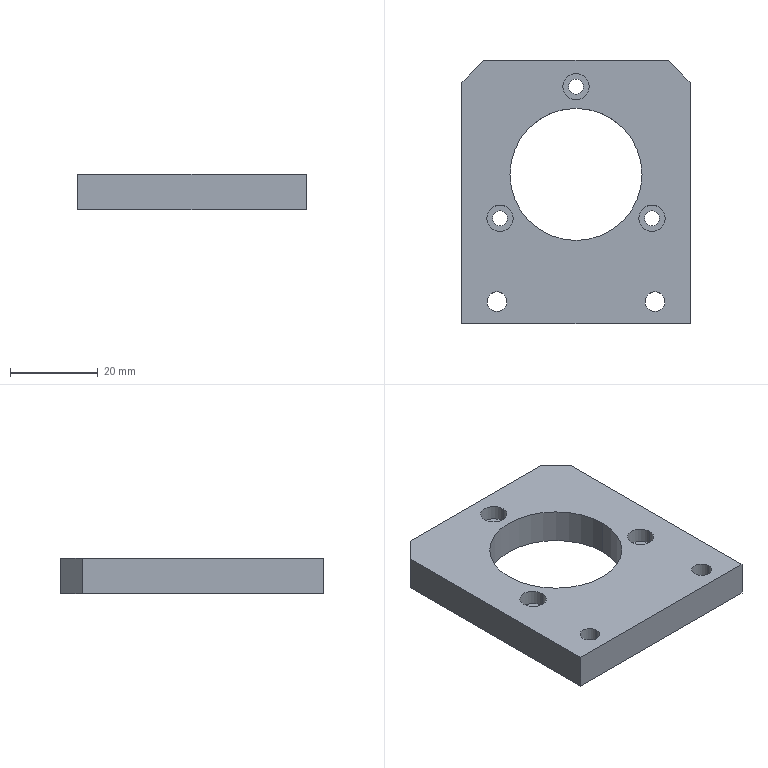Component | SolidWorks | LD101-02--Q1057-Q1-2-1 | 1 solid | 35 faces | box 52 x 60 x 8 mm | volume 18083 mm3 | cylinder 22 | plane 13 | commonest cylinder face diameters 6 x6 3.4 x6 8 x4 4.5 x4 30.1 x2 | material AL6061
build123d program:
from build123d import *

# Parameters (mm, degrees)
SKETCH1_W                                          = 52
SKETCH1_H                                          = 60
BOSS_EXTRUDE1_DEPTH                                = 4
SKETCH2_R                                          = 15.05
CUT_EXTRUDE1_DEPTH                                 = 41.497
HOLE_SIZE_FOR_HEX_SOCKET_HEAD_CAP_SCRE_D           = 3.4
HOLE_SIZE_FOR_HEX_SOCKET_HEAD_CAP_SCRE_CBORE_D     = 6
HOLE_SIZE_FOR_HEX_SOCKET_HEAD_CAP_SCRE_CBORE_DEPTH = 3.4
CIRPATTERN1_COUNT                                  = 3
HOLE_SIZE_FOR_HEX_SOCKET_HEAD_CAP_2_D              = 4.5
HOLE_SIZE_FOR_HEX_SOCKET_HEAD_CAP_2_CBORE_D        = 8
HOLE_SIZE_FOR_HEX_SOCKET_HEAD_CAP_2_CBORE_DEPTH    = 4.6
CHAMFER1_SIZE                                      = 5


with BuildPart() as part:
    # Sketch1 → Boss-Extrude1 (new, symmetric)
    with BuildSketch(Plane.XY):
        Rectangle(SKETCH1_W, SKETCH1_H)
    extrude(amount=BOSS_EXTRUDE1_DEPTH, both=True)

    # Sketch2 → Cut-Extrude1 (cut, through all)
    with BuildSketch(Plane.XY.offset(4)):
        with Locations((0, -4)):
            Circle(SKETCH2_R)
    extrude(amount=-CUT_EXTRUDE1_DEPTH, mode=Mode.SUBTRACT)

    # Hole Size _for_ Hex Socket Head Cap Scre (through all)
    with Locations(Plane.XY.offset(4)):
        with Locations((0, -24)):
            hole_size_for_hex_socket_head_cap_scre = CounterBoreHole(HOLE_SIZE_FOR_HEX_SOCKET_HEAD_CAP_SCRE_D / 2, HOLE_SIZE_FOR_HEX_SOCKET_HEAD_CAP_SCRE_CBORE_D / 2, HOLE_SIZE_FOR_HEX_SOCKET_HEAD_CAP_SCRE_CBORE_DEPTH)

    # CirPattern1: Hole Size _for_ Hex Socket Head Cap Scre ×3 about axis
    cirpattern1_axis = Axis((0, -4, 0), (0, 0, 1))
    for i in range(1, CIRPATTERN1_COUNT):
        add(hole_size_for_hex_socket_head_cap_scre.rotate(cirpattern1_axis, i * 360 / CIRPATTERN1_COUNT), mode=Mode.SUBTRACT)

    # Hole Size _for_ Hex Socket Head Cap  2 (through all)
    with Locations(Plane(origin=(0, 0, -4), x_dir=(-1, 0, 0), z_dir=(0, 0, -1))):
        with Locations((-18, 25), (18, 25)):
            CounterBoreHole(HOLE_SIZE_FOR_HEX_SOCKET_HEAD_CAP_2_D / 2, HOLE_SIZE_FOR_HEX_SOCKET_HEAD_CAP_2_CBORE_D / 2, HOLE_SIZE_FOR_HEX_SOCKET_HEAD_CAP_2_CBORE_DEPTH)

    # Chamfer1
    chamfer1_edges = [part.edges().sort_by_distance(p)[0] for p in [
        (26, -30, 0),
        (-26, -30, 0),
    ]]
    chamfer(chamfer1_edges, length=CHAMFER1_SIZE)


solid = part.part

# Placed as in the assembly
solid = solid.moved(Location((121.71, -185.897, -39.743), (0, 0, 180)))
STEP:
#1=CARTESIAN_POINT('',(3.926,-8.303,-1.541));
#2=VERTEX_POINT('',#1);
#3=CARTESIAN_POINT('',(4.241,-8.303,-1.541));
#4=VERTEX_POINT('',#3);
#5=CARTESIAN_POINT('',(4.083,-8.303,-1.541));
#6=DIRECTION('',(0.,-0.,-1.));
#7=DIRECTION('',(1.,0.,0.));
#8=AXIS2_PLACEMENT_3D('',#5,#6,#7);
#9=CIRCLE('',#8,0.1575);
#10=EDGE_CURVE('',#2,#4,#9,.T.);
#11=ORIENTED_EDGE('',*,*,#10,.F.);
#12=CARTESIAN_POINT('',(3.926,-8.303,-1.722));
#13=VERTEX_POINT('',#12);
#14=CARTESIAN_POINT('',(3.926,-8.303,-1.722));
#15=DIRECTION('',(0.,-0.,-1.));
#16=VECTOR('',#15,39.37);
#17=LINE('',#14,#16);
#18=EDGE_CURVE('',#2,#13,#17,.T.);
#19=ORIENTED_EDGE('',*,*,#18,.T.);
#20=CARTESIAN_POINT('',(4.241,-8.303,-1.722));
#21=VERTEX_POINT('',#20);
#22=CARTESIAN_POINT('',(4.083,-8.303,-1.722));
#23=DIRECTION('',(0.,-0.,-1.));
#24=DIRECTION('',(1.,0.,0.));
#25=AXIS2_PLACEMENT_3D('',#22,#23,#24);
#26=CIRCLE('',#25,0.1575);
#27=EDGE_CURVE('',#13,#21,#26,.T.);
#28=ORIENTED_EDGE('',*,*,#27,.T.);
#29=CARTESIAN_POINT('',(4.241,-8.303,-1.722));
#30=DIRECTION('',(0.,-0.,-1.));
#31=VECTOR('',#30,39.37);
#32=LINE('',#29,#31);
#33=EDGE_CURVE('',#4,#21,#32,.T.);
#34=ORIENTED_EDGE('',*,*,#33,.F.);
#35=EDGE_LOOP('',(#11,#19,#28,#34));
#36=FACE_OUTER_BOUND('',#35,.T.);
#37=CARTESIAN_POINT('',(4.083,-8.303,-1.722));
#38=DIRECTION('',(0.,-0.,-1.));
#39=DIRECTION('',(1.,0.,0.));
#40=AXIS2_PLACEMENT_3D('',#37,#38,#39);
#41=CYLINDRICAL_SURFACE('',#40,0.1575);
#42=ADVANCED_FACE('',(#36),#41,.F.);
#43=CARTESIAN_POINT('',(3.994,-8.303,-1.407));
#44=VERTEX_POINT('',#43);
#45=CARTESIAN_POINT('',(4.172,-8.303,-1.407));
#46=VERTEX_POINT('',#45);
#47=CARTESIAN_POINT('',(4.083,-8.303,-1.407));
#48=DIRECTION('',(0.,-0.,-1.));
#49=DIRECTION('',(1.,0.,0.));
#50=AXIS2_PLACEMENT_3D('',#47,#48,#49);
#51=CIRCLE('',#50,0.08858);
#52=EDGE_CURVE('',#44,#46,#51,.T.);
#53=ORIENTED_EDGE('',*,*,#52,.F.);
#54=CARTESIAN_POINT('',(3.994,-8.303,-1.541));
#55=VERTEX_POINT('',#54);
#56=CARTESIAN_POINT('',(3.994,-8.303,-1.722));
#57=DIRECTION('',(0.,-0.,-1.));
#58=VECTOR('',#57,39.37);
#59=LINE('',#56,#58);
#60=EDGE_CURVE('',#44,#55,#59,.T.);
#61=ORIENTED_EDGE('',*,*,#60,.T.);
#62=CARTESIAN_POINT('',(4.172,-8.303,-1.541));
#63=VERTEX_POINT('',#62);
#64=CARTESIAN_POINT('',(4.083,-8.303,-1.541));
#65=DIRECTION('',(0.,-0.,-1.));
#66=DIRECTION('',(1.,0.,0.));
#67=AXIS2_PLACEMENT_3D('',#64,#65,#66);
#68=CIRCLE('',#67,0.08858);
#69=EDGE_CURVE('',#55,#63,#68,.T.);
#70=ORIENTED_EDGE('',*,*,#69,.T.);
#71=CARTESIAN_POINT('',(4.172,-8.303,-1.722));
#72=DIRECTION('',(0.,-0.,-1.));
#73=VECTOR('',#72,39.37);
#74=LINE('',#71,#73);
#75=EDGE_CURVE('',#46,#63,#74,.T.);
#76=ORIENTED_EDGE('',*,*,#75,.F.);
#77=EDGE_LOOP('',(#53,#61,#70,#76));
#78=FACE_OUTER_BOUND('',#77,.T.);
#79=CARTESIAN_POINT('',(4.083,-8.303,-1.722));
#80=DIRECTION('',(0.,-0.,-1.));
#81=DIRECTION('',(1.,0.,0.));
#82=AXIS2_PLACEMENT_3D('',#79,#80,#81);
#83=CYLINDRICAL_SURFACE('',#82,0.08858);
#84=ADVANCED_FACE('',(#78),#83,.F.);
#85=CARTESIAN_POINT('',(5.343,-8.303,-1.541));
#86=VERTEX_POINT('',#85);
#87=CARTESIAN_POINT('',(5.658,-8.303,-1.541));
#88=VERTEX_POINT('',#87);
#89=CARTESIAN_POINT('',(5.5,-8.303,-1.541));
#90=DIRECTION('',(0.,-0.,-1.));
#91=DIRECTION('',(1.,0.,0.));
#92=AXIS2_PLACEMENT_3D('',#89,#90,#91);
#93=CIRCLE('',#92,0.1575);
#94=EDGE_CURVE('',#86,#88,#93,.T.);
#95=ORIENTED_EDGE('',*,*,#94,.F.);
#96=CARTESIAN_POINT('',(5.343,-8.303,-1.722));
#97=VERTEX_POINT('',#96);
#98=CARTESIAN_POINT('',(5.343,-8.303,-1.722));
#99=DIRECTION('',(0.,-0.,-1.));
#100=VECTOR('',#99,39.37);
#101=LINE('',#98,#100);
#102=EDGE_CURVE('',#86,#97,#101,.T.);
#103=ORIENTED_EDGE('',*,*,#102,.T.);
#104=CARTESIAN_POINT('',(5.658,-8.303,-1.722));
#105=VERTEX_POINT('',#104);
#106=CARTESIAN_POINT('',(5.5,-8.303,-1.722));
#107=DIRECTION('',(0.,-0.,-1.));
#108=DIRECTION('',(1.,0.,0.));
#109=AXIS2_PLACEMENT_3D('',#106,#107,#108);
#110=CIRCLE('',#109,0.1575);
#111=EDGE_CURVE('',#97,#105,#110,.T.);
#112=ORIENTED_EDGE('',*,*,#111,.T.);
#113=CARTESIAN_POINT('',(5.658,-8.303,-1.722));
#114=DIRECTION('',(0.,-0.,-1.));
#115=VECTOR('',#114,39.37);
#116=LINE('',#113,#115);
#117=EDGE_CURVE('',#88,#105,#116,.T.);
#118=ORIENTED_EDGE('',*,*,#117,.F.);
#119=EDGE_LOOP('',(#95,#103,#112,#118));
#120=FACE_OUTER_BOUND('',#119,.T.);
#121=CARTESIAN_POINT('',(5.5,-8.303,-1.722));
#122=DIRECTION('',(0.,-0.,-1.));
#123=DIRECTION('',(1.,0.,0.));
#124=AXIS2_PLACEMENT_3D('',#121,#122,#123);
#125=CYLINDRICAL_SURFACE('',#124,0.1575);
#126=ADVANCED_FACE('',(#120),#125,.F.);
#127=CARTESIAN_POINT('',(5.412,-8.303,-1.407));
#128=VERTEX_POINT('',#127);
#129=CARTESIAN_POINT('',(5.589,-8.303,-1.407));
#130=VERTEX_POINT('',#129);
#131=CARTESIAN_POINT('',(5.5,-8.303,-1.407));
#132=DIRECTION('',(0.,-0.,-1.));
#133=DIRECTION('',(1.,0.,0.));
#134=AXIS2_PLACEMENT_3D('',#131,#132,#133);
#135=CIRCLE('',#134,0.08858);
#136=EDGE_CURVE('',#128,#130,#135,.T.);
#137=ORIENTED_EDGE('',*,*,#136,.F.);
#138=CARTESIAN_POINT('',(5.412,-8.303,-1.541));
#139=VERTEX_POINT('',#138);
#140=CARTESIAN_POINT('',(5.412,-8.303,-1.722));
#141=DIRECTION('',(0.,-0.,-1.));
#142=VECTOR('',#141,39.37);
#143=LINE('',#140,#142);
#144=EDGE_CURVE('',#128,#139,#143,.T.);
#145=ORIENTED_EDGE('',*,*,#144,.T.);
#146=CARTESIAN_POINT('',(5.589,-8.303,-1.541));
#147=VERTEX_POINT('',#146);
#148=CARTESIAN_POINT('',(5.5,-8.303,-1.541));
#149=DIRECTION('',(0.,-0.,-1.));
#150=DIRECTION('',(1.,0.,0.));
#151=AXIS2_PLACEMENT_3D('',#148,#149,#150);
#152=CIRCLE('',#151,0.08858);
#153=EDGE_CURVE('',#139,#147,#152,.T.);
#154=ORIENTED_EDGE('',*,*,#153,.T.);
#155=CARTESIAN_POINT('',(5.589,-8.303,-1.722));
#156=DIRECTION('',(0.,-0.,-1.));
#157=VECTOR('',#156,39.37);
#158=LINE('',#155,#157);
#159=EDGE_CURVE('',#130,#147,#158,.T.);
#160=ORIENTED_EDGE('',*,*,#159,.F.);
#161=EDGE_LOOP('',(#137,#145,#154,#160));
#162=FACE_OUTER_BOUND('',#161,.T.);
#163=CARTESIAN_POINT('',(5.5,-8.303,-1.722));
#164=DIRECTION('',(0.,-0.,-1.));
#165=DIRECTION('',(1.,0.,0.));
#166=AXIS2_PLACEMENT_3D('',#163,#164,#165);
#167=CYLINDRICAL_SURFACE('',#166,0.08858);
#168=ADVANCED_FACE('',(#162),#167,.F.);
#169=CARTESIAN_POINT('',(5.592,-7.555,-1.541));
#170=VERTEX_POINT('',#169);
#171=CARTESIAN_POINT('',(5.356,-7.555,-1.541));
#172=VERTEX_POINT('',#171);
#173=CARTESIAN_POINT('',(5.474,-7.555,-1.541));
#174=DIRECTION('',(-0.,0.,1.));
#175=DIRECTION('',(-1.,0.,0.));
#176=AXIS2_PLACEMENT_3D('',#173,#174,#175);
#177=CIRCLE('',#176,0.1181);
#178=EDGE_CURVE('',#170,#172,#177,.T.);
#179=ORIENTED_EDGE('',*,*,#178,.F.);
#180=CARTESIAN_POINT('',(5.592,-7.555,-1.407));
#181=VERTEX_POINT('',#180);
#182=CARTESIAN_POINT('',(5.592,-7.555,-1.407));
#183=DIRECTION('',(-0.,0.,1.));
#184=VECTOR('',#183,39.37);
#185=LINE('',#182,#184);
#186=EDGE_CURVE('',#170,#181,#185,.T.);
#187=ORIENTED_EDGE('',*,*,#186,.T.);
#188=CARTESIAN_POINT('',(5.356,-7.555,-1.407));
#189=VERTEX_POINT('',#188);
#190=CARTESIAN_POINT('',(5.474,-7.555,-1.407));
#191=DIRECTION('',(-0.,0.,1.));
#192=DIRECTION('',(-1.,0.,0.));
#193=AXIS2_PLACEMENT_3D('',#190,#191,#192);
#194=CIRCLE('',#193,0.1181);
#195=EDGE_CURVE('',#181,#189,#194,.T.);
#196=ORIENTED_EDGE('',*,*,#195,.T.);
#197=CARTESIAN_POINT('',(5.356,-7.555,-1.407));
#198=DIRECTION('',(-0.,0.,1.));
#199=VECTOR('',#198,39.37);
#200=LINE('',#197,#199);
#201=EDGE_CURVE('',#172,#189,#200,.T.);
#202=ORIENTED_EDGE('',*,*,#201,.F.);
#203=EDGE_LOOP('',(#179,#187,#196,#202));
#204=FACE_OUTER_BOUND('',#203,.T.);
#205=CARTESIAN_POINT('',(5.474,-7.555,-1.407));
#206=DIRECTION('',(-0.,0.,1.));
#207=DIRECTION('',(-1.,0.,0.));
#208=AXIS2_PLACEMENT_3D('',#205,#206,#207);
#209=CYLINDRICAL_SURFACE('',#208,0.1181);
#210=ADVANCED_FACE('',(#204),#209,.F.);
#211=CARTESIAN_POINT('',(5.541,-7.555,-1.722));
#212=VERTEX_POINT('',#211);
#213=CARTESIAN_POINT('',(5.407,-7.555,-1.722));
#214=VERTEX_POINT('',#213);
#215=CARTESIAN_POINT('',(5.474,-7.555,-1.722));
#216=DIRECTION('',(-0.,0.,1.));
#217=DIRECTION('',(-1.,0.,0.));
#218=AXIS2_PLACEMENT_3D('',#215,#216,#217);
#219=CIRCLE('',#218,0.06693);
#220=EDGE_CURVE('',#212,#214,#219,.T.);
#221=ORIENTED_EDGE('',*,*,#220,.F.);
#222=CARTESIAN_POINT('',(5.541,-7.555,-1.541));
#223=VERTEX_POINT('',#222);
#224=CARTESIAN_POINT('',(5.541,-7.555,-1.407));
#225=DIRECTION('',(-0.,0.,1.));
#226=VECTOR('',#225,39.37);
#227=LINE('',#224,#226);
#228=EDGE_CURVE('',#212,#223,#227,.T.);
#229=ORIENTED_EDGE('',*,*,#228,.T.);
#230=CARTESIAN_POINT('',(5.407,-7.555,-1.541));
#231=VERTEX_POINT('',#230);
#232=CARTESIAN_POINT('',(5.474,-7.555,-1.541));
#233=DIRECTION('',(-0.,0.,1.));
#234=DIRECTION('',(-1.,0.,0.));
#235=AXIS2_PLACEMENT_3D('',#232,#233,#234);
#236=CIRCLE('',#235,0.06693);
#237=EDGE_CURVE('',#223,#231,#236,.T.);
#238=ORIENTED_EDGE('',*,*,#237,.T.);
#239=CARTESIAN_POINT('',(5.407,-7.555,-1.407));
#240=DIRECTION('',(-0.,0.,1.));
#241=VECTOR('',#240,39.37);
#242=LINE('',#239,#241);
#243=EDGE_CURVE('',#214,#231,#242,.T.);
#244=ORIENTED_EDGE('',*,*,#243,.F.);
#245=EDGE_LOOP('',(#221,#229,#238,#244));
#246=FACE_OUTER_BOUND('',#245,.T.);
#247=CARTESIAN_POINT('',(5.474,-7.555,-1.407));
#248=DIRECTION('',(-0.,0.,1.));
#249=DIRECTION('',(-1.,0.,0.));
#250=AXIS2_PLACEMENT_3D('',#247,#248,#249);
#251=CYLINDRICAL_SURFACE('',#250,0.06693);
#252=ADVANCED_FACE('',(#246),#251,.F.);
#253=CARTESIAN_POINT('',(4.228,-7.555,-1.541));
#254=VERTEX_POINT('',#253);
#255=CARTESIAN_POINT('',(3.992,-7.555,-1.541));
#256=VERTEX_POINT('',#255);
#257=CARTESIAN_POINT('',(4.11,-7.555,-1.541));
#258=DIRECTION('',(-0.,0.,1.));
#259=DIRECTION('',(-1.,0.,0.));
#260=AXIS2_PLACEMENT_3D('',#257,#258,#259);
#261=CIRCLE('',#260,0.1181);
#262=EDGE_CURVE('',#254,#256,#261,.T.);
#263=ORIENTED_EDGE('',*,*,#262,.F.);
#264=CARTESIAN_POINT('',(4.228,-7.555,-1.407));
#265=VERTEX_POINT('',#264);
#266=CARTESIAN_POINT('',(4.228,-7.555,-1.407));
#267=DIRECTION('',(-0.,0.,1.));
#268=VECTOR('',#267,39.37);
#269=LINE('',#266,#268);
#270=EDGE_CURVE('',#254,#265,#269,.T.);
#271=ORIENTED_EDGE('',*,*,#270,.T.);
#272=CARTESIAN_POINT('',(3.992,-7.555,-1.407));
#273=VERTEX_POINT('',#272);
#274=CARTESIAN_POINT('',(4.11,-7.555,-1.407));
#275=DIRECTION('',(-0.,0.,1.));
#276=DIRECTION('',(-1.,0.,0.));
#277=AXIS2_PLACEMENT_3D('',#274,#275,#276);
#278=CIRCLE('',#277,0.1181);
#279=EDGE_CURVE('',#265,#273,#278,.T.);
#280=ORIENTED_EDGE('',*,*,#279,.T.);
#281=CARTESIAN_POINT('',(3.992,-7.555,-1.407));
#282=DIRECTION('',(-0.,0.,1.));
#283=VECTOR('',#282,39.37);
#284=LINE('',#281,#283);
#285=EDGE_CURVE('',#256,#273,#284,.T.);
#286=ORIENTED_EDGE('',*,*,#285,.F.);
#287=EDGE_LOOP('',(#263,#271,#280,#286));
#288=FACE_OUTER_BOUND('',#287,.T.);
#289=CARTESIAN_POINT('',(4.11,-7.555,-1.407));
#290=DIRECTION('',(-0.,0.,1.));
#291=DIRECTION('',(-1.,0.,0.));
#292=AXIS2_PLACEMENT_3D('',#289,#290,#291);
#293=CYLINDRICAL_SURFACE('',#292,0.1181);
#294=ADVANCED_FACE('',(#288),#293,.F.);
#295=CARTESIAN_POINT('',(4.177,-7.555,-1.722));
#296=VERTEX_POINT('',#295);
#297=CARTESIAN_POINT('',(4.043,-7.555,-1.722));
#298=VERTEX_POINT('',#297);
#299=CARTESIAN_POINT('',(4.11,-7.555,-1.722));
#300=DIRECTION('',(-0.,0.,1.));
#301=DIRECTION('',(-1.,0.,0.));
#302=AXIS2_PLACEMENT_3D('',#299,#300,#301);
#303=CIRCLE('',#302,0.06693);
#304=EDGE_CURVE('',#296,#298,#303,.T.);
#305=ORIENTED_EDGE('',*,*,#304,.F.);
#306=CARTESIAN_POINT('',(4.177,-7.555,-1.541));
#307=VERTEX_POINT('',#306);
#308=CARTESIAN_POINT('',(4.177,-7.555,-1.407));
#309=DIRECTION('',(-0.,0.,1.));
#310=VECTOR('',#309,39.37);
#311=LINE('',#308,#310);
#312=EDGE_CURVE('',#296,#307,#311,.T.);
#313=ORIENTED_EDGE('',*,*,#312,.T.);
#314=CARTESIAN_POINT('',(4.043,-7.555,-1.541));
#315=VERTEX_POINT('',#314);
#316=CARTESIAN_POINT('',(4.11,-7.555,-1.541));
#317=DIRECTION('',(-0.,0.,1.));
#318=DIRECTION('',(-1.,0.,0.));
#319=AXIS2_PLACEMENT_3D('',#316,#317,#318);
#320=CIRCLE('',#319,0.06693);
#321=EDGE_CURVE('',#307,#315,#320,.T.);
#322=ORIENTED_EDGE('',*,*,#321,.T.);
#323=CARTESIAN_POINT('',(4.043,-7.555,-1.407));
#324=DIRECTION('',(-0.,0.,1.));
#325=VECTOR('',#324,39.37);
#326=LINE('',#323,#325);
#327=EDGE_CURVE('',#298,#315,#326,.T.);
#328=ORIENTED_EDGE('',*,*,#327,.F.);
#329=EDGE_LOOP('',(#305,#313,#322,#328));
#330=FACE_OUTER_BOUND('',#329,.T.);
#331=CARTESIAN_POINT('',(4.11,-7.555,-1.407));
#332=DIRECTION('',(-0.,0.,1.));
#333=DIRECTION('',(-1.,0.,0.));
#334=AXIS2_PLACEMENT_3D('',#331,#332,#333);
#335=CYLINDRICAL_SURFACE('',#334,0.06693);
#336=ADVANCED_FACE('',(#330),#335,.F.);
#337=CARTESIAN_POINT('',(4.91,-6.374,-1.541));
#338=VERTEX_POINT('',#337);
#339=CARTESIAN_POINT('',(4.674,-6.374,-1.541));
#340=VERTEX_POINT('',#339);
#341=CARTESIAN_POINT('',(4.792,-6.374,-1.541));
#342=DIRECTION('',(-0.,0.,1.));
#343=DIRECTION('',(-1.,0.,0.));
#344=AXIS2_PLACEMENT_3D('',#341,#342,#343);
#345=CIRCLE('',#344,0.1181);
#346=EDGE_CURVE('',#338,#340,#345,.T.);
#347=ORIENTED_EDGE('',*,*,#346,.F.);
#348=CARTESIAN_POINT('',(4.91,-6.374,-1.407));
#349=VERTEX_POINT('',#348);
#350=CARTESIAN_POINT('',(4.91,-6.374,-1.407));
#351=DIRECTION('',(-0.,0.,1.));
#352=VECTOR('',#351,39.37);
#353=LINE('',#350,#352);
#354=EDGE_CURVE('',#338,#349,#353,.T.);
#355=ORIENTED_EDGE('',*,*,#354,.T.);
#356=CARTESIAN_POINT('',(4.674,-6.374,-1.407));
#357=VERTEX_POINT('',#356);
#358=CARTESIAN_POINT('',(4.792,-6.374,-1.407));
#359=DIRECTION('',(-0.,0.,1.));
#360=DIRECTION('',(-1.,0.,0.));
#361=AXIS2_PLACEMENT_3D('',#358,#359,#360);
#362=CIRCLE('',#361,0.1181);
#363=EDGE_CURVE('',#349,#357,#362,.T.);
#364=ORIENTED_EDGE('',*,*,#363,.T.);
#365=CARTESIAN_POINT('',(4.674,-6.374,-1.407));
#366=DIRECTION('',(-0.,0.,1.));
#367=VECTOR('',#366,39.37);
#368=LINE('',#365,#367);
#369=EDGE_CURVE('',#340,#357,#368,.T.);
#370=ORIENTED_EDGE('',*,*,#369,.F.);
#371=EDGE_LOOP('',(#347,#355,#364,#370));
#372=FACE_OUTER_BOUND('',#371,.T.);
#373=CARTESIAN_POINT('',(4.792,-6.374,-1.407));
#374=DIRECTION('',(-0.,0.,1.));
#375=DIRECTION('',(-1.,0.,0.));
#376=AXIS2_PLACEMENT_3D('',#373,#374,#375);
#377=CYLINDRICAL_SURFACE('',#376,0.1181);
#378=ADVANCED_FACE('',(#372),#377,.F.);
#379=CARTESIAN_POINT('',(4.859,-6.374,-1.722));
#380=VERTEX_POINT('',#379);
#381=CARTESIAN_POINT('',(4.725,-6.374,-1.722));
#382=VERTEX_POINT('',#381);
#383=CARTESIAN_POINT('',(4.792,-6.374,-1.722));
#384=DIRECTION('',(-0.,0.,1.));
#385=DIRECTION('',(-1.,0.,0.));
#386=AXIS2_PLACEMENT_3D('',#383,#384,#385);
#387=CIRCLE('',#386,0.06693);
#388=EDGE_CURVE('',#380,#382,#387,.T.);
#389=ORIENTED_EDGE('',*,*,#388,.F.);
#390=CARTESIAN_POINT('',(4.859,-6.374,-1.541));
#391=VERTEX_POINT('',#390);
#392=CARTESIAN_POINT('',(4.859,-6.374,-1.407));
#393=DIRECTION('',(-0.,0.,1.));
#394=VECTOR('',#393,39.37);
#395=LINE('',#392,#394);
#396=EDGE_CURVE('',#380,#391,#395,.T.);
#397=ORIENTED_EDGE('',*,*,#396,.T.);
#398=CARTESIAN_POINT('',(4.725,-6.374,-1.541));
#399=VERTEX_POINT('',#398);
#400=CARTESIAN_POINT('',(4.792,-6.374,-1.541));
#401=DIRECTION('',(-0.,0.,1.));
#402=DIRECTION('',(-1.,0.,0.));
#403=AXIS2_PLACEMENT_3D('',#400,#401,#402);
#404=CIRCLE('',#403,0.06693);
#405=EDGE_CURVE('',#391,#399,#404,.T.);
#406=ORIENTED_EDGE('',*,*,#405,.T.);
#407=CARTESIAN_POINT('',(4.725,-6.374,-1.407));
#408=DIRECTION('',(-0.,0.,1.));
#409=VECTOR('',#408,39.37);
#410=LINE('',#407,#409);
#411=EDGE_CURVE('',#382,#399,#410,.T.);
#412=ORIENTED_EDGE('',*,*,#411,.F.);
#413=EDGE_LOOP('',(#389,#397,#406,#412));
#414=FACE_OUTER_BOUND('',#413,.T.);
#415=CARTESIAN_POINT('',(4.792,-6.374,-1.407));
#416=DIRECTION('',(-0.,0.,1.));
#417=DIRECTION('',(-1.,0.,0.));
#418=AXIS2_PLACEMENT_3D('',#415,#416,#417);
#419=CYLINDRICAL_SURFACE('',#418,0.06693);
#420=ADVANCED_FACE('',(#414),#419,.F.);
#421=CARTESIAN_POINT('',(5.384,-7.161,-1.722));
#422=VERTEX_POINT('',#421);
#423=CARTESIAN_POINT('',(4.199,-7.161,-1.722));
#424=VERTEX_POINT('',#423);
#425=CARTESIAN_POINT('',(4.792,-7.161,-1.722));
#426=DIRECTION('',(-0.,0.,1.));
#427=DIRECTION('',(-1.,0.,0.));
#428=AXIS2_PLACEMENT_3D('',#425,#426,#427);
#429=CIRCLE('',#428,0.5925);
#430=EDGE_CURVE('',#422,#424,#429,.T.);
#431=ORIENTED_EDGE('',*,*,#430,.F.);
#432=CARTESIAN_POINT('',(5.384,-7.161,-1.407));
#433=VERTEX_POINT('',#432);
#434=CARTESIAN_POINT('',(5.384,-7.161,-1.722));
#435=DIRECTION('',(-0.,0.,1.));
#436=VECTOR('',#435,39.37);
#437=LINE('',#434,#436);
#438=EDGE_CURVE('',#422,#433,#437,.T.);
#439=ORIENTED_EDGE('',*,*,#438,.T.);
#440=CARTESIAN_POINT('',(4.199,-7.161,-1.407));
#441=VERTEX_POINT('',#440);
#442=CARTESIAN_POINT('',(4.792,-7.161,-1.407));
#443=DIRECTION('',(-0.,0.,1.));
#444=DIRECTION('',(-1.,0.,0.));
#445=AXIS2_PLACEMENT_3D('',#442,#443,#444);
#446=CIRCLE('',#445,0.5925);
#447=EDGE_CURVE('',#433,#441,#446,.T.);
#448=ORIENTED_EDGE('',*,*,#447,.T.);
#449=CARTESIAN_POINT('',(4.199,-7.161,-1.722));
#450=DIRECTION('',(-0.,0.,1.));
#451=VECTOR('',#450,39.37);
#452=LINE('',#449,#451);
#453=EDGE_CURVE('',#424,#441,#452,.T.);
#454=ORIENTED_EDGE('',*,*,#453,.F.);
#455=EDGE_LOOP('',(#431,#439,#448,#454));
#456=FACE_OUTER_BOUND('',#455,.T.);
#457=CARTESIAN_POINT('',(4.792,-7.161,-1.722));
#458=DIRECTION('',(-0.,0.,1.));
#459=DIRECTION('',(-1.,0.,0.));
#460=AXIS2_PLACEMENT_3D('',#457,#458,#459);
#461=CYLINDRICAL_SURFACE('',#460,0.5925);
#462=ADVANCED_FACE('',(#456),#461,.F.);
#463=CARTESIAN_POINT('',(3.768,-6.335,-1.407));
#464=VERTEX_POINT('',#463);
#465=CARTESIAN_POINT('',(3.768,-8.5,-1.407));
#466=VERTEX_POINT('',#465);
#467=CARTESIAN_POINT('',(3.768,-6.138,-1.407));
#468=DIRECTION('',(0.,-1.,0.));
#469=VECTOR('',#468,39.37);
#470=LINE('',#467,#469);
#471=EDGE_CURVE('',#464,#466,#470,.T.);
#472=ORIENTED_EDGE('',*,*,#471,.F.);
#473=CARTESIAN_POINT('',(3.768,-6.335,-1.722));
#474=VERTEX_POINT('',#473);
#475=CARTESIAN_POINT('',(3.768,-6.335,-1.407));
#476=DIRECTION('',(0.,-0.,-1.));
#477=VECTOR('',#476,39.37);
#478=LINE('',#475,#477);
#479=EDGE_CURVE('',#464,#474,#478,.T.);
#480=ORIENTED_EDGE('',*,*,#479,.T.);
#481=CARTESIAN_POINT('',(3.768,-8.5,-1.722));
#482=VERTEX_POINT('',#481);
#483=CARTESIAN_POINT('',(3.768,-6.138,-1.722));
#484=DIRECTION('',(0.,-1.,0.));
#485=VECTOR('',#484,39.37);
#486=LINE('',#483,#485);
#487=EDGE_CURVE('',#474,#482,#486,.T.);
#488=ORIENTED_EDGE('',*,*,#487,.T.);
#489=CARTESIAN_POINT('',(3.768,-8.5,-1.407));
#490=DIRECTION('',(0.,-0.,-1.));
#491=VECTOR('',#490,39.37);
#492=LINE('',#489,#491);
#493=EDGE_CURVE('',#466,#482,#492,.T.);
#494=ORIENTED_EDGE('',*,*,#493,.F.);
#495=EDGE_LOOP('',(#472,#480,#488,#494));
#496=FACE_OUTER_BOUND('',#495,.T.);
#497=CARTESIAN_POINT('',(3.768,-6.138,-1.407));
#498=DIRECTION('',(1.,0.,0.));
#499=DIRECTION('',(-0.,0.,1.));
#500=AXIS2_PLACEMENT_3D('',#497,#498,#499);
#501=PLANE('',#500);
#502=ADVANCED_FACE('',(#496),#501,.F.);
#503=CARTESIAN_POINT('',(5.815,-8.5,-1.722));
#504=VERTEX_POINT('',#503);
#505=CARTESIAN_POINT('',(5.815,-8.5,-1.722));
#506=DIRECTION('',(1.,0.,0.));
#507=VECTOR('',#506,39.37);
#508=LINE('',#505,#507);
#509=EDGE_CURVE('',#482,#504,#508,.T.);
#510=ORIENTED_EDGE('',*,*,#509,.T.);
#511=CARTESIAN_POINT('',(5.815,-8.5,-1.407));
#512=VERTEX_POINT('',#511);
#513=CARTESIAN_POINT('',(5.815,-8.5,-1.407));
#514=DIRECTION('',(0.,-0.,-1.));
#515=VECTOR('',#514,39.37);
#516=LINE('',#513,#515);
#517=EDGE_CURVE('',#512,#504,#516,.T.);
#518=ORIENTED_EDGE('',*,*,#517,.F.);
#519=CARTESIAN_POINT('',(5.815,-8.5,-1.407));
#520=DIRECTION('',(1.,0.,0.));
#521=VECTOR('',#520,39.37);
#522=LINE('',#519,#521);
#523=EDGE_CURVE('',#466,#512,#522,.T.);
#524=ORIENTED_EDGE('',*,*,#523,.F.);
#525=ORIENTED_EDGE('',*,*,#493,.T.);
#526=EDGE_LOOP('',(#510,#518,#524,#525));
#527=FACE_OUTER_BOUND('',#526,.T.);
#528=CARTESIAN_POINT('',(5.815,-8.5,-1.407));
#529=DIRECTION('',(-0.,1.,-0.));
#530=DIRECTION('',(0.,-0.,-1.));
#531=AXIS2_PLACEMENT_3D('',#528,#529,#530);
#532=PLANE('',#531);
#533=ADVANCED_FACE('',(#527),#532,.F.);
#534=CARTESIAN_POINT('',(5.815,-6.335,-1.722));
#535=VERTEX_POINT('',#534);
#536=CARTESIAN_POINT('',(5.815,-6.138,-1.722));
#537=DIRECTION('',(-0.,1.,-0.));
#538=VECTOR('',#537,39.37);
#539=LINE('',#536,#538);
#540=EDGE_CURVE('',#504,#535,#539,.T.);
#541=ORIENTED_EDGE('',*,*,#540,.T.);
#542=CARTESIAN_POINT('',(5.815,-6.335,-1.407));
#543=VERTEX_POINT('',#542);
#544=CARTESIAN_POINT('',(5.815,-6.335,-1.407));
#545=DIRECTION('',(-0.,0.,1.));
#546=VECTOR('',#545,39.37);
#547=LINE('',#544,#546);
#548=EDGE_CURVE('',#535,#543,#547,.T.);
#549=ORIENTED_EDGE('',*,*,#548,.T.);
#550=CARTESIAN_POINT('',(5.815,-6.138,-1.407));
#551=DIRECTION('',(-0.,1.,-0.));
#552=VECTOR('',#551,39.37);
#553=LINE('',#550,#552);
#554=EDGE_CURVE('',#512,#543,#553,.T.);
#555=ORIENTED_EDGE('',*,*,#554,.F.);
#556=ORIENTED_EDGE('',*,*,#517,.T.);
#557=EDGE_LOOP('',(#541,#549,#555,#556));
#558=FACE_OUTER_BOUND('',#557,.T.);
#559=CARTESIAN_POINT('',(5.815,-6.138,-1.407));
#560=DIRECTION('',(-1.,-0.,-0.));
#561=DIRECTION('',(0.,-0.,-1.));
#562=AXIS2_PLACEMENT_3D('',#559,#560,#561);
#563=PLANE('',#562);
#564=ADVANCED_FACE('',(#558),#563,.F.);
#565=CARTESIAN_POINT('',(5.619,-6.138,-1.407));
#566=VERTEX_POINT('',#565);
#567=CARTESIAN_POINT('',(3.965,-6.138,-1.407));
#568=VERTEX_POINT('',#567);
#569=CARTESIAN_POINT('',(5.815,-6.138,-1.407));
#570=DIRECTION('',(-1.,-0.,-0.));
#571=VECTOR('',#570,39.37);
#572=LINE('',#569,#571);
#573=EDGE_CURVE('',#566,#568,#572,.T.);
#574=ORIENTED_EDGE('',*,*,#573,.F.);
#575=CARTESIAN_POINT('',(5.619,-6.138,-1.722));
#576=VERTEX_POINT('',#575);
#577=CARTESIAN_POINT('',(5.619,-6.138,-1.407));
#578=DIRECTION('',(0.,-0.,-1.));
#579=VECTOR('',#578,39.37);
#580=LINE('',#577,#579);
#581=EDGE_CURVE('',#566,#576,#580,.T.);
#582=ORIENTED_EDGE('',*,*,#581,.T.);
#583=CARTESIAN_POINT('',(3.965,-6.138,-1.722));
#584=VERTEX_POINT('',#583);
#585=CARTESIAN_POINT('',(5.815,-6.138,-1.722));
#586=DIRECTION('',(-1.,-0.,-0.));
#587=VECTOR('',#586,39.37);
#588=LINE('',#585,#587);
#589=EDGE_CURVE('',#576,#584,#588,.T.);
#590=ORIENTED_EDGE('',*,*,#589,.T.);
#591=CARTESIAN_POINT('',(3.965,-6.138,-1.407));
#592=DIRECTION('',(-0.,0.,1.));
#593=VECTOR('',#592,39.37);
#594=LINE('',#591,#593);
#595=EDGE_CURVE('',#584,#568,#594,.T.);
#596=ORIENTED_EDGE('',*,*,#595,.T.);
#597=EDGE_LOOP('',(#574,#582,#590,#596));
#598=FACE_OUTER_BOUND('',#597,.T.);
#599=CARTESIAN_POINT('',(5.815,-6.138,-1.407));
#600=DIRECTION('',(0.,-1.,0.));
#601=DIRECTION('',(-0.,0.,1.));
#602=AXIS2_PLACEMENT_3D('',#599,#600,#601);
#603=PLANE('',#602);
#604=ADVANCED_FACE('',(#598),#603,.F.);
#605=CARTESIAN_POINT('',(4.083,-8.303,-1.407));
#606=DIRECTION('',(0.,-0.,-1.));
#607=DIRECTION('',(1.,0.,0.));
#608=AXIS2_PLACEMENT_3D('',#605,#606,#607);
#609=CIRCLE('',#608,0.08858);
#610=EDGE_CURVE('',#46,#44,#609,.T.);
#611=ORIENTED_EDGE('',*,*,#610,.T.);
#612=ORIENTED_EDGE('',*,*,#52,.T.);
#613=EDGE_LOOP('',(#611,#612));
#614=FACE_BOUND('',#613,.T.);
#615=CARTESIAN_POINT('',(5.5,-8.303,-1.407));
#616=DIRECTION('',(0.,-0.,-1.));
#617=DIRECTION('',(1.,0.,0.));
#618=AXIS2_PLACEMENT_3D('',#615,#616,#617);
#619=CIRCLE('',#618,0.08858);
#620=EDGE_CURVE('',#130,#128,#619,.T.);
#621=ORIENTED_EDGE('',*,*,#620,.T.);
#622=ORIENTED_EDGE('',*,*,#136,.T.);
#623=EDGE_LOOP('',(#621,#622));
#624=FACE_BOUND('',#623,.T.);
#625=CARTESIAN_POINT('',(5.474,-7.555,-1.407));
#626=DIRECTION('',(-0.,0.,1.));
#627=DIRECTION('',(-1.,0.,0.));
#628=AXIS2_PLACEMENT_3D('',#625,#626,#627);
#629=CIRCLE('',#628,0.1181);
#630=EDGE_CURVE('',#189,#181,#629,.T.);
#631=ORIENTED_EDGE('',*,*,#630,.F.);
#632=ORIENTED_EDGE('',*,*,#195,.F.);
#633=EDGE_LOOP('',(#631,#632));
#634=FACE_BOUND('',#633,.T.);
#635=CARTESIAN_POINT('',(4.11,-7.555,-1.407));
#636=DIRECTION('',(-0.,0.,1.));
#637=DIRECTION('',(-1.,0.,0.));
#638=AXIS2_PLACEMENT_3D('',#635,#636,#637);
#639=CIRCLE('',#638,0.1181);
#640=EDGE_CURVE('',#273,#265,#639,.T.);
#641=ORIENTED_EDGE('',*,*,#640,.F.);
#642=ORIENTED_EDGE('',*,*,#279,.F.);
#643=EDGE_LOOP('',(#641,#642));
#644=FACE_BOUND('',#643,.T.);
#645=CARTESIAN_POINT('',(4.792,-6.374,-1.407));
#646=DIRECTION('',(-0.,0.,1.));
#647=DIRECTION('',(-1.,0.,0.));
#648=AXIS2_PLACEMENT_3D('',#645,#646,#647);
#649=CIRCLE('',#648,0.1181);
#650=EDGE_CURVE('',#357,#349,#649,.T.);
#651=ORIENTED_EDGE('',*,*,#650,.F.);
#652=ORIENTED_EDGE('',*,*,#363,.F.);
#653=EDGE_LOOP('',(#651,#652));
#654=FACE_BOUND('',#653,.T.);
#655=CARTESIAN_POINT('',(4.792,-7.161,-1.407));
#656=DIRECTION('',(-0.,0.,1.));
#657=DIRECTION('',(-1.,0.,0.));
#658=AXIS2_PLACEMENT_3D('',#655,#656,#657);
#659=CIRCLE('',#658,0.5925);
#660=EDGE_CURVE('',#441,#433,#659,.T.);
#661=ORIENTED_EDGE('',*,*,#660,.F.);
#662=ORIENTED_EDGE('',*,*,#447,.F.);
#663=EDGE_LOOP('',(#661,#662));
#664=FACE_BOUND('',#663,.T.);
#665=ORIENTED_EDGE('',*,*,#554,.T.);
#666=CARTESIAN_POINT('',(5.619,-6.138,-1.407));
#667=DIRECTION('',(-0.7071,0.7071,-0.));
#668=VECTOR('',#667,39.37);
#669=LINE('',#666,#668);
#670=EDGE_CURVE('',#543,#566,#669,.T.);
#671=ORIENTED_EDGE('',*,*,#670,.T.);
#672=ORIENTED_EDGE('',*,*,#573,.T.);
#673=CARTESIAN_POINT('',(3.768,-6.335,-1.407));
#674=DIRECTION('',(-0.7071,-0.7071,-0.));
#675=VECTOR('',#674,39.37);
#676=LINE('',#673,#675);
#677=EDGE_CURVE('',#568,#464,#676,.T.);
#678=ORIENTED_EDGE('',*,*,#677,.T.);
#679=ORIENTED_EDGE('',*,*,#471,.T.);
#680=ORIENTED_EDGE('',*,*,#523,.T.);
#681=EDGE_LOOP('',(#665,#671,#672,#678,#679,#680));
#682=FACE_OUTER_BOUND('',#681,.T.);
#683=CARTESIAN_POINT('',(4.792,-7.319,-1.407));
#684=DIRECTION('',(0.,-0.,-1.));
#685=DIRECTION('',(1.,0.,0.));
#686=AXIS2_PLACEMENT_3D('',#683,#684,#685);
#687=PLANE('',#686);
#688=ADVANCED_FACE('',(#614,#624,#634,#644,#654,#664,#682),#687,.F.);
#689=CARTESIAN_POINT('',(4.083,-8.303,-1.722));
#690=DIRECTION('',(0.,-0.,-1.));
#691=DIRECTION('',(1.,0.,0.));
#692=AXIS2_PLACEMENT_3D('',#689,#690,#691);
#693=CIRCLE('',#692,0.1575);
#694=EDGE_CURVE('',#21,#13,#693,.T.);
#695=ORIENTED_EDGE('',*,*,#694,.F.);
#696=ORIENTED_EDGE('',*,*,#27,.F.);
#697=EDGE_LOOP('',(#695,#696));
#698=FACE_BOUND('',#697,.T.);
#699=CARTESIAN_POINT('',(5.5,-8.303,-1.722));
#700=DIRECTION('',(0.,-0.,-1.));
#701=DIRECTION('',(1.,0.,0.));
#702=AXIS2_PLACEMENT_3D('',#699,#700,#701);
#703=CIRCLE('',#702,0.1575);
#704=EDGE_CURVE('',#105,#97,#703,.T.);
#705=ORIENTED_EDGE('',*,*,#704,.F.);
#706=ORIENTED_EDGE('',*,*,#111,.F.);
#707=EDGE_LOOP('',(#705,#706));
#708=FACE_BOUND('',#707,.T.);
#709=CARTESIAN_POINT('',(5.474,-7.555,-1.722));
#710=DIRECTION('',(-0.,0.,1.));
#711=DIRECTION('',(-1.,0.,0.));
#712=AXIS2_PLACEMENT_3D('',#709,#710,#711);
#713=CIRCLE('',#712,0.06693);
#714=EDGE_CURVE('',#214,#212,#713,.T.);
#715=ORIENTED_EDGE('',*,*,#714,.T.);
#716=ORIENTED_EDGE('',*,*,#220,.T.);
#717=EDGE_LOOP('',(#715,#716));
#718=FACE_BOUND('',#717,.T.);
#719=CARTESIAN_POINT('',(4.11,-7.555,-1.722));
#720=DIRECTION('',(-0.,0.,1.));
#721=DIRECTION('',(-1.,0.,0.));
#722=AXIS2_PLACEMENT_3D('',#719,#720,#721);
#723=CIRCLE('',#722,0.06693);
#724=EDGE_CURVE('',#298,#296,#723,.T.);
#725=ORIENTED_EDGE('',*,*,#724,.T.);
#726=ORIENTED_EDGE('',*,*,#304,.T.);
#727=EDGE_LOOP('',(#725,#726));
#728=FACE_BOUND('',#727,.T.);
#729=CARTESIAN_POINT('',(4.792,-6.374,-1.722));
#730=DIRECTION('',(-0.,0.,1.));
#731=DIRECTION('',(-1.,0.,0.));
#732=AXIS2_PLACEMENT_3D('',#729,#730,#731);
#733=CIRCLE('',#732,0.06693);
#734=EDGE_CURVE('',#382,#380,#733,.T.);
#735=ORIENTED_EDGE('',*,*,#734,.T.);
#736=ORIENTED_EDGE('',*,*,#388,.T.);
#737=EDGE_LOOP('',(#735,#736));
#738=FACE_BOUND('',#737,.T.);
#739=CARTESIAN_POINT('',(4.792,-7.161,-1.722));
#740=DIRECTION('',(-0.,0.,1.));
#741=DIRECTION('',(-1.,0.,0.));
#742=AXIS2_PLACEMENT_3D('',#739,#740,#741);
#743=CIRCLE('',#742,0.5925);
#744=EDGE_CURVE('',#424,#422,#743,.T.);
#745=ORIENTED_EDGE('',*,*,#744,.T.);
#746=ORIENTED_EDGE('',*,*,#430,.T.);
#747=EDGE_LOOP('',(#745,#746));
#748=FACE_BOUND('',#747,.T.);
#749=ORIENTED_EDGE('',*,*,#589,.F.);
#750=CARTESIAN_POINT('',(5.796,-6.315,-1.722));
#751=DIRECTION('',(0.7071,-0.7071,0.));
#752=VECTOR('',#751,39.37);
#753=LINE('',#750,#752);
#754=EDGE_CURVE('',#576,#535,#753,.T.);
#755=ORIENTED_EDGE('',*,*,#754,.T.);
#756=ORIENTED_EDGE('',*,*,#540,.F.);
#757=ORIENTED_EDGE('',*,*,#509,.F.);
#758=ORIENTED_EDGE('',*,*,#487,.F.);
#759=CARTESIAN_POINT('',(3.788,-6.315,-1.722));
#760=DIRECTION('',(0.7071,0.7071,0.));
#761=VECTOR('',#760,39.37);
#762=LINE('',#759,#761);
#763=EDGE_CURVE('',#474,#584,#762,.T.);
#764=ORIENTED_EDGE('',*,*,#763,.T.);
#765=EDGE_LOOP('',(#749,#755,#756,#757,#758,#764));
#766=FACE_OUTER_BOUND('',#765,.T.);
#767=CARTESIAN_POINT('',(4.792,-7.319,-1.722));
#768=DIRECTION('',(0.,-0.,-1.));
#769=DIRECTION('',(1.,0.,0.));
#770=AXIS2_PLACEMENT_3D('',#767,#768,#769);
#771=PLANE('',#770);
#772=ADVANCED_FACE('',(#698,#708,#718,#728,#738,#748,#766),#771,.T.);
#773=ORIENTED_EDGE('',*,*,#438,.F.);
#774=ORIENTED_EDGE('',*,*,#744,.F.);
#775=ORIENTED_EDGE('',*,*,#453,.T.);
#776=ORIENTED_EDGE('',*,*,#660,.T.);
#777=EDGE_LOOP('',(#773,#774,#775,#776));
#778=FACE_OUTER_BOUND('',#777,.T.);
#779=CARTESIAN_POINT('',(4.792,-7.161,-1.722));
#780=DIRECTION('',(-0.,0.,1.));
#781=DIRECTION('',(-1.,0.,0.));
#782=AXIS2_PLACEMENT_3D('',#779,#780,#781);
#783=CYLINDRICAL_SURFACE('',#782,0.5925);
#784=ADVANCED_FACE('',(#778),#783,.F.);
#785=ORIENTED_EDGE('',*,*,#396,.F.);
#786=ORIENTED_EDGE('',*,*,#734,.F.);
#787=ORIENTED_EDGE('',*,*,#411,.T.);
#788=CARTESIAN_POINT('',(4.792,-6.374,-1.541));
#789=DIRECTION('',(-0.,0.,1.));
#790=DIRECTION('',(-1.,0.,0.));
#791=AXIS2_PLACEMENT_3D('',#788,#789,#790);
#792=CIRCLE('',#791,0.06693);
#793=EDGE_CURVE('',#399,#391,#792,.T.);
#794=ORIENTED_EDGE('',*,*,#793,.T.);
#795=EDGE_LOOP('',(#785,#786,#787,#794));
#796=FACE_OUTER_BOUND('',#795,.T.);
#797=CARTESIAN_POINT('',(4.792,-6.374,-1.407));
#798=DIRECTION('',(-0.,0.,1.));
#799=DIRECTION('',(-1.,0.,0.));
#800=AXIS2_PLACEMENT_3D('',#797,#798,#799);
#801=CYLINDRICAL_SURFACE('',#800,0.06693);
#802=ADVANCED_FACE('',(#796),#801,.F.);
#803=ORIENTED_EDGE('',*,*,#793,.F.);
#804=ORIENTED_EDGE('',*,*,#405,.F.);
#805=EDGE_LOOP('',(#803,#804));
#806=FACE_BOUND('',#805,.T.);
#807=CARTESIAN_POINT('',(4.792,-6.374,-1.541));
#808=DIRECTION('',(-0.,0.,1.));
#809=DIRECTION('',(-1.,0.,0.));
#810=AXIS2_PLACEMENT_3D('',#807,#808,#809);
#811=CIRCLE('',#810,0.1181);
#812=EDGE_CURVE('',#340,#338,#811,.T.);
#813=ORIENTED_EDGE('',*,*,#812,.T.);
#814=ORIENTED_EDGE('',*,*,#346,.T.);
#815=EDGE_LOOP('',(#813,#814));
#816=FACE_OUTER_BOUND('',#815,.T.);
#817=CARTESIAN_POINT('',(4.725,-6.374,-1.541));
#818=DIRECTION('',(0.,-0.,-1.));
#819=DIRECTION('',(1.,0.,0.));
#820=AXIS2_PLACEMENT_3D('',#817,#818,#819);
#821=PLANE('',#820);
#822=ADVANCED_FACE('',(#806,#816),#821,.F.);
#823=ORIENTED_EDGE('',*,*,#354,.F.);
#824=ORIENTED_EDGE('',*,*,#812,.F.);
#825=ORIENTED_EDGE('',*,*,#369,.T.);
#826=ORIENTED_EDGE('',*,*,#650,.T.);
#827=EDGE_LOOP('',(#823,#824,#825,#826));
#828=FACE_OUTER_BOUND('',#827,.T.);
#829=CARTESIAN_POINT('',(4.792,-6.374,-1.407));
#830=DIRECTION('',(-0.,0.,1.));
#831=DIRECTION('',(-1.,0.,0.));
#832=AXIS2_PLACEMENT_3D('',#829,#830,#831);
#833=CYLINDRICAL_SURFACE('',#832,0.1181);
#834=ADVANCED_FACE('',(#828),#833,.F.);
#835=ORIENTED_EDGE('',*,*,#312,.F.);
#836=ORIENTED_EDGE('',*,*,#724,.F.);
#837=ORIENTED_EDGE('',*,*,#327,.T.);
#838=CARTESIAN_POINT('',(4.11,-7.555,-1.541));
#839=DIRECTION('',(-0.,0.,1.));
#840=DIRECTION('',(-1.,0.,0.));
#841=AXIS2_PLACEMENT_3D('',#838,#839,#840);
#842=CIRCLE('',#841,0.06693);
#843=EDGE_CURVE('',#315,#307,#842,.T.);
#844=ORIENTED_EDGE('',*,*,#843,.T.);
#845=EDGE_LOOP('',(#835,#836,#837,#844));
#846=FACE_OUTER_BOUND('',#845,.T.);
#847=CARTESIAN_POINT('',(4.11,-7.555,-1.407));
#848=DIRECTION('',(-0.,0.,1.));
#849=DIRECTION('',(-1.,0.,0.));
#850=AXIS2_PLACEMENT_3D('',#847,#848,#849);
#851=CYLINDRICAL_SURFACE('',#850,0.06693);
#852=ADVANCED_FACE('',(#846),#851,.F.);
#853=ORIENTED_EDGE('',*,*,#843,.F.);
#854=ORIENTED_EDGE('',*,*,#321,.F.);
#855=EDGE_LOOP('',(#853,#854));
#856=FACE_BOUND('',#855,.T.);
#857=CARTESIAN_POINT('',(4.11,-7.555,-1.541));
#858=DIRECTION('',(-0.,0.,1.));
#859=DIRECTION('',(-1.,0.,0.));
#860=AXIS2_PLACEMENT_3D('',#857,#858,#859);
#861=CIRCLE('',#860,0.1181);
#862=EDGE_CURVE('',#256,#254,#861,.T.);
#863=ORIENTED_EDGE('',*,*,#862,.T.);
#864=ORIENTED_EDGE('',*,*,#262,.T.);
#865=EDGE_LOOP('',(#863,#864));
#866=FACE_OUTER_BOUND('',#865,.T.);
#867=CARTESIAN_POINT('',(4.043,-7.555,-1.541));
#868=DIRECTION('',(0.,-0.,-1.));
#869=DIRECTION('',(1.,0.,0.));
#870=AXIS2_PLACEMENT_3D('',#867,#868,#869);
#871=PLANE('',#870);
#872=ADVANCED_FACE('',(#856,#866),#871,.F.);
#873=ORIENTED_EDGE('',*,*,#270,.F.);
#874=ORIENTED_EDGE('',*,*,#862,.F.);
#875=ORIENTED_EDGE('',*,*,#285,.T.);
#876=ORIENTED_EDGE('',*,*,#640,.T.);
#877=EDGE_LOOP('',(#873,#874,#875,#876));
#878=FACE_OUTER_BOUND('',#877,.T.);
#879=CARTESIAN_POINT('',(4.11,-7.555,-1.407));
#880=DIRECTION('',(-0.,0.,1.));
#881=DIRECTION('',(-1.,0.,0.));
#882=AXIS2_PLACEMENT_3D('',#879,#880,#881);
#883=CYLINDRICAL_SURFACE('',#882,0.1181);
#884=ADVANCED_FACE('',(#878),#883,.F.);
#885=ORIENTED_EDGE('',*,*,#228,.F.);
#886=ORIENTED_EDGE('',*,*,#714,.F.);
#887=ORIENTED_EDGE('',*,*,#243,.T.);
#888=CARTESIAN_POINT('',(5.474,-7.555,-1.541));
#889=DIRECTION('',(-0.,0.,1.));
#890=DIRECTION('',(-1.,0.,0.));
#891=AXIS2_PLACEMENT_3D('',#888,#889,#890);
#892=CIRCLE('',#891,0.06693);
#893=EDGE_CURVE('',#231,#223,#892,.T.);
#894=ORIENTED_EDGE('',*,*,#893,.T.);
#895=EDGE_LOOP('',(#885,#886,#887,#894));
#896=FACE_OUTER_BOUND('',#895,.T.);
#897=CARTESIAN_POINT('',(5.474,-7.555,-1.407));
#898=DIRECTION('',(-0.,0.,1.));
#899=DIRECTION('',(-1.,0.,0.));
#900=AXIS2_PLACEMENT_3D('',#897,#898,#899);
#901=CYLINDRICAL_SURFACE('',#900,0.06693);
#902=ADVANCED_FACE('',(#896),#901,.F.);
#903=ORIENTED_EDGE('',*,*,#893,.F.);
#904=ORIENTED_EDGE('',*,*,#237,.F.);
#905=EDGE_LOOP('',(#903,#904));
#906=FACE_BOUND('',#905,.T.);
#907=CARTESIAN_POINT('',(5.474,-7.555,-1.541));
#908=DIRECTION('',(-0.,0.,1.));
#909=DIRECTION('',(-1.,0.,0.));
#910=AXIS2_PLACEMENT_3D('',#907,#908,#909);
#911=CIRCLE('',#910,0.1181);
#912=EDGE_CURVE('',#172,#170,#911,.T.);
#913=ORIENTED_EDGE('',*,*,#912,.T.);
#914=ORIENTED_EDGE('',*,*,#178,.T.);
#915=EDGE_LOOP('',(#913,#914));
#916=FACE_OUTER_BOUND('',#915,.T.);
#917=CARTESIAN_POINT('',(5.407,-7.555,-1.541));
#918=DIRECTION('',(0.,-0.,-1.));
#919=DIRECTION('',(1.,0.,0.));
#920=AXIS2_PLACEMENT_3D('',#917,#918,#919);
#921=PLANE('',#920);
#922=ADVANCED_FACE('',(#906,#916),#921,.F.);
#923=ORIENTED_EDGE('',*,*,#186,.F.);
#924=ORIENTED_EDGE('',*,*,#912,.F.);
#925=ORIENTED_EDGE('',*,*,#201,.T.);
#926=ORIENTED_EDGE('',*,*,#630,.T.);
#927=EDGE_LOOP('',(#923,#924,#925,#926));
#928=FACE_OUTER_BOUND('',#927,.T.);
#929=CARTESIAN_POINT('',(5.474,-7.555,-1.407));
#930=DIRECTION('',(-0.,0.,1.));
#931=DIRECTION('',(-1.,0.,0.));
#932=AXIS2_PLACEMENT_3D('',#929,#930,#931);
#933=CYLINDRICAL_SURFACE('',#932,0.1181);
#934=ADVANCED_FACE('',(#928),#933,.F.);
#935=ORIENTED_EDGE('',*,*,#144,.F.);
#936=ORIENTED_EDGE('',*,*,#620,.F.);
#937=ORIENTED_EDGE('',*,*,#159,.T.);
#938=CARTESIAN_POINT('',(5.5,-8.303,-1.541));
#939=DIRECTION('',(0.,-0.,-1.));
#940=DIRECTION('',(1.,0.,0.));
#941=AXIS2_PLACEMENT_3D('',#938,#939,#940);
#942=CIRCLE('',#941,0.08858);
#943=EDGE_CURVE('',#147,#139,#942,.T.);
#944=ORIENTED_EDGE('',*,*,#943,.T.);
#945=EDGE_LOOP('',(#935,#936,#937,#944));
#946=FACE_OUTER_BOUND('',#945,.T.);
#947=CARTESIAN_POINT('',(5.5,-8.303,-1.722));
#948=DIRECTION('',(0.,-0.,-1.));
#949=DIRECTION('',(1.,0.,0.));
#950=AXIS2_PLACEMENT_3D('',#947,#948,#949);
#951=CYLINDRICAL_SURFACE('',#950,0.08858);
#952=ADVANCED_FACE('',(#946),#951,.F.);
#953=ORIENTED_EDGE('',*,*,#943,.F.);
#954=ORIENTED_EDGE('',*,*,#153,.F.);
#955=EDGE_LOOP('',(#953,#954));
#956=FACE_BOUND('',#955,.T.);
#957=CARTESIAN_POINT('',(5.5,-8.303,-1.541));
#958=DIRECTION('',(0.,-0.,-1.));
#959=DIRECTION('',(1.,0.,0.));
#960=AXIS2_PLACEMENT_3D('',#957,#958,#959);
#961=CIRCLE('',#960,0.1575);
#962=EDGE_CURVE('',#88,#86,#961,.T.);
#963=ORIENTED_EDGE('',*,*,#962,.T.);
#964=ORIENTED_EDGE('',*,*,#94,.T.);
#965=EDGE_LOOP('',(#963,#964));
#966=FACE_OUTER_BOUND('',#965,.T.);
#967=CARTESIAN_POINT('',(5.412,-8.303,-1.541));
#968=DIRECTION('',(-0.,0.,1.));
#969=DIRECTION('',(-1.,-0.,-0.));
#970=AXIS2_PLACEMENT_3D('',#967,#968,#969);
#971=PLANE('',#970);
#972=ADVANCED_FACE('',(#956,#966),#971,.F.);
#973=ORIENTED_EDGE('',*,*,#102,.F.);
#974=ORIENTED_EDGE('',*,*,#962,.F.);
#975=ORIENTED_EDGE('',*,*,#117,.T.);
#976=ORIENTED_EDGE('',*,*,#704,.T.);
#977=EDGE_LOOP('',(#973,#974,#975,#976));
#978=FACE_OUTER_BOUND('',#977,.T.);
#979=CARTESIAN_POINT('',(5.5,-8.303,-1.722));
#980=DIRECTION('',(0.,-0.,-1.));
#981=DIRECTION('',(1.,0.,0.));
#982=AXIS2_PLACEMENT_3D('',#979,#980,#981);
#983=CYLINDRICAL_SURFACE('',#982,0.1575);
#984=ADVANCED_FACE('',(#978),#983,.F.);
#985=ORIENTED_EDGE('',*,*,#60,.F.);
#986=ORIENTED_EDGE('',*,*,#610,.F.);
#987=ORIENTED_EDGE('',*,*,#75,.T.);
#988=CARTESIAN_POINT('',(4.083,-8.303,-1.541));
#989=DIRECTION('',(0.,-0.,-1.));
#990=DIRECTION('',(1.,0.,0.));
#991=AXIS2_PLACEMENT_3D('',#988,#989,#990);
#992=CIRCLE('',#991,0.08858);
#993=EDGE_CURVE('',#63,#55,#992,.T.);
#994=ORIENTED_EDGE('',*,*,#993,.T.);
#995=EDGE_LOOP('',(#985,#986,#987,#994));
#996=FACE_OUTER_BOUND('',#995,.T.);
#997=CARTESIAN_POINT('',(4.083,-8.303,-1.722));
#998=DIRECTION('',(0.,-0.,-1.));
#999=DIRECTION('',(1.,0.,0.));
#1000=AXIS2_PLACEMENT_3D('',#997,#998,#999);
#1001=CYLINDRICAL_SURFACE('',#1000,0.08858);
#1002=ADVANCED_FACE('',(#996),#1001,.F.);
#1003=ORIENTED_EDGE('',*,*,#993,.F.);
#1004=ORIENTED_EDGE('',*,*,#69,.F.);
#1005=EDGE_LOOP('',(#1003,#1004));
#1006=FACE_BOUND('',#1005,.T.);
#1007=CARTESIAN_POINT('',(4.083,-8.303,-1.541));
#1008=DIRECTION('',(0.,-0.,-1.));
#1009=DIRECTION('',(1.,0.,0.));
#1010=AXIS2_PLACEMENT_3D('',#1007,#1008,#1009);
#1011=CIRCLE('',#1010,0.1575);
#1012=EDGE_CURVE('',#4,#2,#1011,.T.);
#1013=ORIENTED_EDGE('',*,*,#1012,.T.);
#1014=ORIENTED_EDGE('',*,*,#10,.T.);
#1015=EDGE_LOOP('',(#1013,#1014));
#1016=FACE_OUTER_BOUND('',#1015,.T.);
#1017=CARTESIAN_POINT('',(3.994,-8.303,-1.541));
#1018=DIRECTION('',(-0.,0.,1.));
#1019=DIRECTION('',(-1.,-0.,-0.));
#1020=AXIS2_PLACEMENT_3D('',#1017,#1018,#1019);
#1021=PLANE('',#1020);
#1022=ADVANCED_FACE('',(#1006,#1016),#1021,.F.);
#1023=ORIENTED_EDGE('',*,*,#18,.F.);
#1024=ORIENTED_EDGE('',*,*,#1012,.F.);
#1025=ORIENTED_EDGE('',*,*,#33,.T.);
#1026=ORIENTED_EDGE('',*,*,#694,.T.);
#1027=EDGE_LOOP('',(#1023,#1024,#1025,#1026));
#1028=FACE_OUTER_BOUND('',#1027,.T.);
#1029=CARTESIAN_POINT('',(4.083,-8.303,-1.722));
#1030=DIRECTION('',(0.,-0.,-1.));
#1031=DIRECTION('',(1.,0.,0.));
#1032=AXIS2_PLACEMENT_3D('',#1029,#1030,#1031);
#1033=CYLINDRICAL_SURFACE('',#1032,0.1575);
#1034=ADVANCED_FACE('',(#1028),#1033,.F.);
#1035=ORIENTED_EDGE('',*,*,#670,.F.);
#1036=ORIENTED_EDGE('',*,*,#548,.F.);
#1037=ORIENTED_EDGE('',*,*,#754,.F.);
#1038=ORIENTED_EDGE('',*,*,#581,.F.);
#1039=EDGE_LOOP('',(#1035,#1036,#1037,#1038));
#1040=FACE_OUTER_BOUND('',#1039,.T.);
#1041=CARTESIAN_POINT('',(5.619,-6.138,-1.407));
#1042=DIRECTION('',(-0.7071,-0.7071,-0.));
#1043=DIRECTION('',(0.,-0.,-1.));
#1044=AXIS2_PLACEMENT_3D('',#1041,#1042,#1043);
#1045=PLANE('',#1044);
#1046=ADVANCED_FACE('',(#1040),#1045,.F.);
#1047=ORIENTED_EDGE('',*,*,#677,.F.);
#1048=ORIENTED_EDGE('',*,*,#595,.F.);
#1049=ORIENTED_EDGE('',*,*,#763,.F.);
#1050=ORIENTED_EDGE('',*,*,#479,.F.);
#1051=EDGE_LOOP('',(#1047,#1048,#1049,#1050));
#1052=FACE_OUTER_BOUND('',#1051,.T.);
#1053=CARTESIAN_POINT('',(3.768,-6.335,-1.407));
#1054=DIRECTION('',(0.7071,-0.7071,0.));
#1055=DIRECTION('',(0.,-0.,-1.));
#1056=AXIS2_PLACEMENT_3D('',#1053,#1054,#1055);
#1057=PLANE('',#1056);
#1058=ADVANCED_FACE('',(#1052),#1057,.F.);
#1059=CLOSED_SHELL('',(#42,#84,#126,#168,#210,#252,#294,#336,#378,#420,#462,#502,#533,#564,#604,#688,#772,#784,#802,#822,#834,#852,#872,#884,#902,#922,#934,#952,#972,#984,#1002,#1022,#1034,#1046,#1058));
#1060=MANIFOLD_SOLID_BREP('',#1059);
#1061=CARTESIAN_POINT('',(0.,0.,0.));
#1062=DIRECTION('',(0.,0.,1.));
#1063=DIRECTION('',(1.,0.,0.));
#1064=AXIS2_PLACEMENT_3D('',#1061,#1062,#1063);
#1065=(LENGTH_UNIT()NAMED_UNIT(*)SI_UNIT($,.METRE.));
#1066=LENGTH_MEASURE_WITH_UNIT(LENGTH_MEASURE(0.0254),#1065);
#1067=DIMENSIONAL_EXPONENTS(1.,0.,0.,0.,0.,0.,0.);
#1068=(CONVERSION_BASED_UNIT('',#1066)LENGTH_UNIT()NAMED_UNIT(#1067));
#1069=UNCERTAINTY_MEASURE_WITH_UNIT(LENGTH_MEASURE(0.00001),#1068,'','');
#1070=(NAMED_UNIT(*)PLANE_ANGLE_UNIT()SI_UNIT($,.RADIAN.));
#1071=(NAMED_UNIT(*)SI_UNIT($,.STERADIAN.)SOLID_ANGLE_UNIT());
#1072=(GEOMETRIC_REPRESENTATION_CONTEXT(3)GLOBAL_UNCERTAINTY_ASSIGNED_CONTEXT((#1069))GLOBAL_UNIT_ASSIGNED_CONTEXT((#1068,#1070,#1071))REPRESENTATION_CONTEXT('',''));
#1073=ADVANCED_BREP_SHAPE_REPRESENTATION('',(#1060,#1064),#1072);
#1074=COLOUR_RGB('',0.7922,0.8196,0.9333);
#1075=FILL_AREA_STYLE_COLOUR('',#1074);
#1076=FILL_AREA_STYLE('',(#1075));
#1077=SURFACE_STYLE_FILL_AREA(#1076);
#1078=SURFACE_SIDE_STYLE('',(#1077));
#1079=SURFACE_STYLE_USAGE(.BOTH.,#1078);
#1080=PRESENTATION_STYLE_ASSIGNMENT((#1079));
#1081=STYLED_ITEM('',(#1080),#1060);
#1082=(LENGTH_UNIT()NAMED_UNIT(*)SI_UNIT($,.METRE.));
#1083=LENGTH_MEASURE_WITH_UNIT(LENGTH_MEASURE(0.0254),#1082);
#1084=DIMENSIONAL_EXPONENTS(1.,0.,0.,0.,0.,0.,0.);
#1085=(CONVERSION_BASED_UNIT('',#1083)LENGTH_UNIT()NAMED_UNIT(#1084));
#1086=UNCERTAINTY_MEASURE_WITH_UNIT(LENGTH_MEASURE(0.00001),#1085,'','');
#1087=(NAMED_UNIT(*)PLANE_ANGLE_UNIT()SI_UNIT($,.RADIAN.));
#1088=(NAMED_UNIT(*)SI_UNIT($,.STERADIAN.)SOLID_ANGLE_UNIT());
#1089=(GEOMETRIC_REPRESENTATION_CONTEXT(3)GLOBAL_UNCERTAINTY_ASSIGNED_CONTEXT((#1086))GLOBAL_UNIT_ASSIGNED_CONTEXT((#1085,#1087,#1088))REPRESENTATION_CONTEXT('',''));
#1090=MECHANICAL_DESIGN_GEOMETRIC_PRESENTATION_REPRESENTATION('',(#1081),#1089);
#1091=PRESENTATION_LAYER_ASSIGNMENT('','',(#1081));